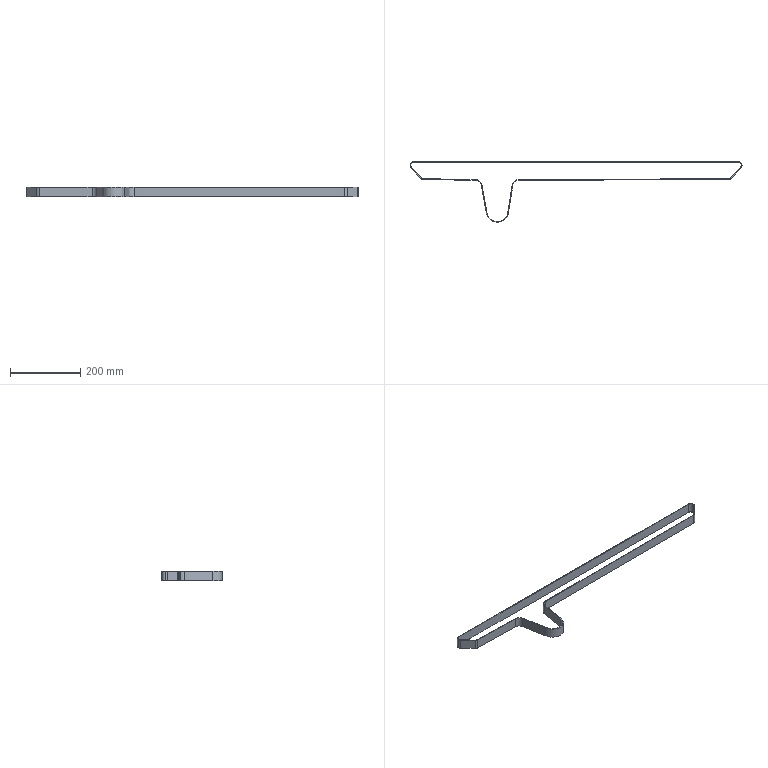Component | SolidWorks | --MA18S20041JR-SHuangGWBelt1-1 | 1 solid | 32 faces | box 946 x 172 x 28 mm | volume 118080 mm3 | cylinder 16 | plane 16 | commonest cylinder face diameters 16 x5 20 x5 30 x2 34 x2 64 x1 60 x1
build123d program:
from build123d import *

# Parameters (mm, degrees)
EXTRUDE_THIN1_DEPTH = 28


with BuildPart() as part:
    # Sketch1 → Extrude-Thin1 (new body)
    with BuildSketch(Plane.XY):
        with BuildLine():
            Line((170.069, -109.183), (163.702, -27.72))
            ThreePointArc((163.702, -27.72), (159.583, -18.516), (150.567, -14))
            Line((150.567, -14), (1.149, 4.256))
            ThreePointArc((1.149, 4.256), (-2.62, 5.511), (-5.603, 8.136))
            Line((-5.603, 8.136), (-30.416, 40.821))
            ThreePointArc((-30.416, 40.821), (-31.17, 51.763), (-21.436, 56.816))
            Line((-21.436, 56.816), (899.788, -37.114))
            ThreePointArc((899.788, -37.114), (908.302, -44.028), (905.354, -54.592))
            Line((905.354, -54.592), (874.455, -81.597))
            ThreePointArc((874.455, -81.597), (870.933, -83.588), (866.91, -84.021))
            Line((866.91, -84.021), (269.576, -26.131))
            ThreePointArc((269.576, -26.131), (259.577, -28.738), (253.636, -37.194))
            Line((253.636, -37.194), (232.89, -114.939))
            ThreePointArc((232.89, -114.939), (199.052, -138.556), (170.069, -109.183))
        make_face()
        with BuildLine():
            Line((172.063, -109.027), (165.696, -27.564))
            ThreePointArc((165.696, -27.564), (161.028, -17.133), (150.81, -12.014))
            Line((150.81, -12.014), (1.392, 6.241))
            ThreePointArc((1.392, 6.241), (-1.624, 7.246), (-4.01, 9.345))
            Line((-4.01, 9.345), (-28.823, 42.03))
            ThreePointArc((-28.823, 42.03), (-29.427, 50.784), (-21.639, 54.826))
            Line((-21.639, 54.826), (899.585, -39.104))
            ThreePointArc((899.585, -39.104), (906.396, -44.635), (904.038, -53.086))
            Line((904.038, -53.086), (873.139, -80.091))
            ThreePointArc((873.139, -80.091), (870.321, -81.684), (867.103, -82.03))
            Line((867.103, -82.03), (269.769, -24.141))
            ThreePointArc((269.769, -24.141), (258.436, -27.095), (251.704, -36.678))
            Line((251.704, -36.678), (230.958, -114.424))
            ThreePointArc((230.958, -114.424), (199.234, -136.564), (172.063, -109.027))
        make_face(mode=Mode.SUBTRACT)
    extrude(amount=EXTRUDE_THIN1_DEPTH)


solid = part.part

# Placed as in the assembly
solid = solid.moved(Location((-138.867, 52.35, 19), (0, 0, 5.822)))
STEP:
#1=CARTESIAN_POINT('',(-6.534,4.122,1.85));
#2=VERTEX_POINT('',#1);
#3=CARTESIAN_POINT('',(-6.847,3.775,1.85));
#4=VERTEX_POINT('',#3);
#5=CARTESIAN_POINT('',(-6.534,3.807,1.85));
#6=DIRECTION('',(0.,0.,1.));
#7=DIRECTION('',(0.9948,0.1014,0.));
#8=AXIS2_PLACEMENT_3D('',#5,#6,#7);
#9=CIRCLE('',#8,0.315);
#10=EDGE_CURVE('',#2,#4,#9,.T.);
#11=ORIENTED_EDGE('',*,*,#10,.T.);
#12=CARTESIAN_POINT('',(-6.847,3.775,0.748));
#13=VERTEX_POINT('',#12);
#14=CARTESIAN_POINT('',(-6.847,3.775,1.85));
#15=DIRECTION('',(0.,0.,-1.));
#16=VECTOR('',#15,39.37);
#17=LINE('',#14,#16);
#18=EDGE_CURVE('',#4,#13,#17,.T.);
#19=ORIENTED_EDGE('',*,*,#18,.T.);
#20=CARTESIAN_POINT('',(-6.534,4.122,0.748));
#21=VERTEX_POINT('',#20);
#22=CARTESIAN_POINT('',(-6.534,3.807,0.748));
#23=DIRECTION('',(0.,0.,1.));
#24=DIRECTION('',(0.9948,0.1014,0.));
#25=AXIS2_PLACEMENT_3D('',#22,#23,#24);
#26=CIRCLE('',#25,0.315);
#27=EDGE_CURVE('',#21,#13,#26,.T.);
#28=ORIENTED_EDGE('',*,*,#27,.F.);
#29=CARTESIAN_POINT('',(-6.534,4.122,1.85));
#30=DIRECTION('',(0.,0.,-1.));
#31=VECTOR('',#30,39.37);
#32=LINE('',#29,#31);
#33=EDGE_CURVE('',#2,#21,#32,.T.);
#34=ORIENTED_EDGE('',*,*,#33,.F.);
#35=EDGE_LOOP('',(#11,#19,#28,#34));
#36=FACE_OUTER_BOUND('',#35,.T.);
#37=CARTESIAN_POINT('',(-6.534,3.807,1.85));
#38=DIRECTION('',(0.,0.,-1.));
#39=DIRECTION('',(-0.9948,-0.1014,0.));
#40=AXIS2_PLACEMENT_3D('',#37,#38,#39);
#41=CYLINDRICAL_SURFACE('',#40,0.315);
#42=ADVANCED_FACE('',(#36),#41,.F.);
#43=CARTESIAN_POINT('',(-6.925,3.767,1.85));
#44=VERTEX_POINT('',#43);
#45=CARTESIAN_POINT('',(-6.822,3.538,1.85));
#46=VERTEX_POINT('',#45);
#47=CARTESIAN_POINT('',(-6.534,3.807,1.85));
#48=DIRECTION('',(0.,0.,1.));
#49=DIRECTION('',(0.9948,0.1014,0.));
#50=AXIS2_PLACEMENT_3D('',#47,#48,#49);
#51=CIRCLE('',#50,0.3937);
#52=EDGE_CURVE('',#44,#46,#51,.T.);
#53=ORIENTED_EDGE('',*,*,#52,.F.);
#54=CARTESIAN_POINT('',(-6.925,3.767,0.748));
#55=VERTEX_POINT('',#54);
#56=CARTESIAN_POINT('',(-6.925,3.767,1.85));
#57=DIRECTION('',(0.,0.,-1.));
#58=VECTOR('',#57,39.37);
#59=LINE('',#56,#58);
#60=EDGE_CURVE('',#44,#55,#59,.T.);
#61=ORIENTED_EDGE('',*,*,#60,.T.);
#62=CARTESIAN_POINT('',(-6.822,3.538,0.748));
#63=VERTEX_POINT('',#62);
#64=CARTESIAN_POINT('',(-6.534,3.807,0.748));
#65=DIRECTION('',(0.,0.,1.));
#66=DIRECTION('',(0.9948,0.1014,0.));
#67=AXIS2_PLACEMENT_3D('',#64,#65,#66);
#68=CIRCLE('',#67,0.3937);
#69=EDGE_CURVE('',#55,#63,#68,.T.);
#70=ORIENTED_EDGE('',*,*,#69,.T.);
#71=CARTESIAN_POINT('',(-6.822,3.538,1.85));
#72=DIRECTION('',(0.,0.,-1.));
#73=VECTOR('',#72,39.37);
#74=LINE('',#71,#73);
#75=EDGE_CURVE('',#46,#63,#74,.T.);
#76=ORIENTED_EDGE('',*,*,#75,.F.);
#77=EDGE_LOOP('',(#53,#61,#70,#76));
#78=FACE_OUTER_BOUND('',#77,.T.);
#79=CARTESIAN_POINT('',(-6.534,3.807,1.85));
#80=DIRECTION('',(0.,0.,-1.));
#81=DIRECTION('',(-0.9948,-0.1014,0.));
#82=AXIS2_PLACEMENT_3D('',#79,#80,#81);
#83=CYLINDRICAL_SURFACE('',#82,0.3937);
#84=ADVANCED_FACE('',(#78),#83,.T.);
#85=CARTESIAN_POINT('',(30.211,3.538,1.85));
#86=VERTEX_POINT('',#85);
#87=CARTESIAN_POINT('',(29.923,4.201,1.85));
#88=VERTEX_POINT('',#87);
#89=CARTESIAN_POINT('',(29.923,3.807,1.85));
#90=DIRECTION('',(0.,0.,1.));
#91=DIRECTION('',(0.9948,0.1014,0.));
#92=AXIS2_PLACEMENT_3D('',#89,#90,#91);
#93=CIRCLE('',#92,0.3937);
#94=EDGE_CURVE('',#86,#88,#93,.T.);
#95=ORIENTED_EDGE('',*,*,#94,.T.);
#96=CARTESIAN_POINT('',(-6.534,4.201,1.85));
#97=VERTEX_POINT('',#96);
#98=CARTESIAN_POINT('',(-6.534,4.201,1.85));
#99=DIRECTION('',(-1.,0.,0.));
#100=VECTOR('',#99,39.37);
#101=LINE('',#98,#100);
#102=EDGE_CURVE('',#88,#97,#101,.T.);
#103=ORIENTED_EDGE('',*,*,#102,.T.);
#104=CARTESIAN_POINT('',(-6.534,3.807,1.85));
#105=DIRECTION('',(0.,0.,1.));
#106=DIRECTION('',(0.9948,0.1014,0.));
#107=AXIS2_PLACEMENT_3D('',#104,#105,#106);
#108=CIRCLE('',#107,0.3937);
#109=EDGE_CURVE('',#97,#44,#108,.T.);
#110=ORIENTED_EDGE('',*,*,#109,.T.);
#111=ORIENTED_EDGE('',*,*,#52,.T.);
#112=CARTESIAN_POINT('',(-5.719,2.357,1.85));
#113=VERTEX_POINT('',#112);
#114=CARTESIAN_POINT('',(-5.719,2.357,1.85));
#115=DIRECTION('',(0.6823,-0.7311,0.));
#116=VECTOR('',#115,39.37);
#117=LINE('',#114,#116);
#118=EDGE_CURVE('',#46,#113,#117,.T.);
#119=ORIENTED_EDGE('',*,*,#118,.T.);
#120=CARTESIAN_POINT('',(-5.439,2.232,1.85));
#121=VERTEX_POINT('',#120);
#122=CARTESIAN_POINT('',(-5.431,2.626,1.85));
#123=DIRECTION('',(0.,0.,1.));
#124=DIRECTION('',(0.9948,0.1014,0.));
#125=AXIS2_PLACEMENT_3D('',#122,#123,#124);
#126=CIRCLE('',#125,0.3937);
#127=EDGE_CURVE('',#113,#121,#126,.T.);
#128=ORIENTED_EDGE('',*,*,#127,.T.);
#129=CARTESIAN_POINT('',(0.486,2.114,1.85));
#130=VERTEX_POINT('',#129);
#131=CARTESIAN_POINT('',(-5.439,2.232,1.85));
#132=DIRECTION('',(0.9998,-0.01996,0.));
#133=VECTOR('',#132,39.37);
#134=LINE('',#131,#133);
#135=EDGE_CURVE('',#121,#130,#134,.T.);
#136=ORIENTED_EDGE('',*,*,#135,.T.);
#137=CARTESIAN_POINT('',(1.055,1.629,1.85));
#138=VERTEX_POINT('',#137);
#139=CARTESIAN_POINT('',(0.4742,1.524,1.85));
#140=DIRECTION('',(0.,0.,-1.));
#141=DIRECTION('',(0.9948,0.1014,0.));
#142=AXIS2_PLACEMENT_3D('',#139,#140,#141);
#143=CIRCLE('',#142,0.5906);
#144=EDGE_CURVE('',#130,#138,#143,.T.);
#145=ORIENTED_EDGE('',*,*,#144,.T.);
#146=CARTESIAN_POINT('',(1.63,-1.536,1.85));
#147=VERTEX_POINT('',#146);
#148=CARTESIAN_POINT('',(1.63,-1.536,1.85));
#149=DIRECTION('',(0.1786,-0.9839,0.));
#150=VECTOR('',#149,39.37);
#151=LINE('',#148,#150);
#152=EDGE_CURVE('',#138,#147,#151,.T.);
#153=ORIENTED_EDGE('',*,*,#152,.T.);
#154=CARTESIAN_POINT('',(4.113,-1.511,1.85));
#155=VERTEX_POINT('',#154);
#156=CARTESIAN_POINT('',(2.869,-1.311,1.85));
#157=DIRECTION('',(0.,0.,1.));
#158=DIRECTION('',(0.9948,0.1014,0.));
#159=AXIS2_PLACEMENT_3D('',#156,#157,#158);
#160=CIRCLE('',#159,1.26);
#161=EDGE_CURVE('',#147,#155,#160,.T.);
#162=ORIENTED_EDGE('',*,*,#161,.T.);
#163=CARTESIAN_POINT('',(4.615,1.617,1.85));
#164=VERTEX_POINT('',#163);
#165=CARTESIAN_POINT('',(4.615,1.617,1.85));
#166=DIRECTION('',(0.1585,0.9874,0.));
#167=VECTOR('',#166,39.37);
#168=LINE('',#165,#167);
#169=EDGE_CURVE('',#155,#164,#168,.T.);
#170=ORIENTED_EDGE('',*,*,#169,.T.);
#171=CARTESIAN_POINT('',(5.196,2.114,1.85));
#172=VERTEX_POINT('',#171);
#173=CARTESIAN_POINT('',(5.199,1.524,1.85));
#174=DIRECTION('',(0.,0.,-1.));
#175=DIRECTION('',(0.9948,0.1014,0.));
#176=AXIS2_PLACEMENT_3D('',#173,#174,#175);
#177=CIRCLE('',#176,0.5906);
#178=EDGE_CURVE('',#164,#172,#177,.T.);
#179=ORIENTED_EDGE('',*,*,#178,.T.);
#180=CARTESIAN_POINT('',(28.823,2.232,1.85));
#181=VERTEX_POINT('',#180);
#182=CARTESIAN_POINT('',(28.823,2.232,1.85));
#183=DIRECTION('',(1.,0.004999,0.));
#184=VECTOR('',#183,39.37);
#185=LINE('',#182,#184);
#186=EDGE_CURVE('',#172,#181,#185,.T.);
#187=ORIENTED_EDGE('',*,*,#186,.T.);
#188=CARTESIAN_POINT('',(29.108,2.357,1.85));
#189=VERTEX_POINT('',#188);
#190=CARTESIAN_POINT('',(28.821,2.626,1.85));
#191=DIRECTION('',(0.,0.,1.));
#192=DIRECTION('',(0.9948,0.1014,0.));
#193=AXIS2_PLACEMENT_3D('',#190,#191,#192);
#194=CIRCLE('',#193,0.3937);
#195=EDGE_CURVE('',#181,#189,#194,.T.);
#196=ORIENTED_EDGE('',*,*,#195,.T.);
#197=CARTESIAN_POINT('',(30.211,3.538,1.85));
#198=DIRECTION('',(0.6823,0.7311,0.));
#199=VECTOR('',#198,39.37);
#200=LINE('',#197,#199);
#201=EDGE_CURVE('',#189,#86,#200,.T.);
#202=ORIENTED_EDGE('',*,*,#201,.T.);
#203=EDGE_LOOP('',(#95,#103,#110,#111,#119,#128,#136,#145,#153,#162,#170,#179,#187,#196,#202));
#204=FACE_OUTER_BOUND('',#203,.T.);
#205=CARTESIAN_POINT('',(29.923,4.122,1.85));
#206=VERTEX_POINT('',#205);
#207=CARTESIAN_POINT('',(-6.534,4.122,1.85));
#208=DIRECTION('',(-1.,0.,0.));
#209=VECTOR('',#208,39.37);
#210=LINE('',#207,#209);
#211=EDGE_CURVE('',#206,#2,#210,.T.);
#212=ORIENTED_EDGE('',*,*,#211,.F.);
#213=CARTESIAN_POINT('',(30.153,3.592,1.85));
#214=VERTEX_POINT('',#213);
#215=CARTESIAN_POINT('',(29.923,3.807,1.85));
#216=DIRECTION('',(0.,0.,1.));
#217=DIRECTION('',(0.9948,0.1014,0.));
#218=AXIS2_PLACEMENT_3D('',#215,#216,#217);
#219=CIRCLE('',#218,0.315);
#220=EDGE_CURVE('',#214,#206,#219,.T.);
#221=ORIENTED_EDGE('',*,*,#220,.F.);
#222=CARTESIAN_POINT('',(29.051,2.411,1.85));
#223=VERTEX_POINT('',#222);
#224=CARTESIAN_POINT('',(30.153,3.592,1.85));
#225=DIRECTION('',(0.6823,0.7311,0.));
#226=VECTOR('',#225,39.37);
#227=LINE('',#224,#226);
#228=EDGE_CURVE('',#223,#214,#227,.T.);
#229=ORIENTED_EDGE('',*,*,#228,.F.);
#230=CARTESIAN_POINT('',(28.822,2.311,1.85));
#231=VERTEX_POINT('',#230);
#232=CARTESIAN_POINT('',(28.821,2.626,1.85));
#233=DIRECTION('',(0.,0.,1.));
#234=DIRECTION('',(0.9948,0.1014,0.));
#235=AXIS2_PLACEMENT_3D('',#232,#233,#234);
#236=CIRCLE('',#235,0.315);
#237=EDGE_CURVE('',#231,#223,#236,.T.);
#238=ORIENTED_EDGE('',*,*,#237,.F.);
#239=CARTESIAN_POINT('',(5.195,2.193,1.85));
#240=VERTEX_POINT('',#239);
#241=CARTESIAN_POINT('',(28.822,2.311,1.85));
#242=DIRECTION('',(1.,0.004999,0.));
#243=VECTOR('',#242,39.37);
#244=LINE('',#241,#243);
#245=EDGE_CURVE('',#240,#231,#244,.T.);
#246=ORIENTED_EDGE('',*,*,#245,.F.);
#247=CARTESIAN_POINT('',(4.538,1.63,1.85));
#248=VERTEX_POINT('',#247);
#249=CARTESIAN_POINT('',(5.199,1.524,1.85));
#250=DIRECTION('',(0.,0.,-1.));
#251=DIRECTION('',(0.9948,0.1014,0.));
#252=AXIS2_PLACEMENT_3D('',#249,#250,#251);
#253=CIRCLE('',#252,0.6693);
#254=EDGE_CURVE('',#248,#240,#253,.T.);
#255=ORIENTED_EDGE('',*,*,#254,.F.);
#256=CARTESIAN_POINT('',(4.036,-1.498,1.85));
#257=VERTEX_POINT('',#256);
#258=CARTESIAN_POINT('',(4.538,1.63,1.85));
#259=DIRECTION('',(0.1585,0.9874,0.));
#260=VECTOR('',#259,39.37);
#261=LINE('',#258,#260);
#262=EDGE_CURVE('',#257,#248,#261,.T.);
#263=ORIENTED_EDGE('',*,*,#262,.F.);
#264=CARTESIAN_POINT('',(1.707,-1.522,1.85));
#265=VERTEX_POINT('',#264);
#266=CARTESIAN_POINT('',(2.869,-1.311,1.85));
#267=DIRECTION('',(0.,0.,1.));
#268=DIRECTION('',(0.9948,0.1014,0.));
#269=AXIS2_PLACEMENT_3D('',#266,#267,#268);
#270=CIRCLE('',#269,1.181);
#271=EDGE_CURVE('',#265,#257,#270,.T.);
#272=ORIENTED_EDGE('',*,*,#271,.F.);
#273=CARTESIAN_POINT('',(1.133,1.643,1.85));
#274=VERTEX_POINT('',#273);
#275=CARTESIAN_POINT('',(1.707,-1.522,1.85));
#276=DIRECTION('',(0.1786,-0.9839,0.));
#277=VECTOR('',#276,39.37);
#278=LINE('',#275,#277);
#279=EDGE_CURVE('',#274,#265,#278,.T.);
#280=ORIENTED_EDGE('',*,*,#279,.F.);
#281=CARTESIAN_POINT('',(0.4875,2.193,1.85));
#282=VERTEX_POINT('',#281);
#283=CARTESIAN_POINT('',(0.4742,1.524,1.85));
#284=DIRECTION('',(0.,0.,-1.));
#285=DIRECTION('',(0.9948,0.1014,0.));
#286=AXIS2_PLACEMENT_3D('',#283,#284,#285);
#287=CIRCLE('',#286,0.6693);
#288=EDGE_CURVE('',#282,#274,#287,.T.);
#289=ORIENTED_EDGE('',*,*,#288,.F.);
#290=CARTESIAN_POINT('',(-5.438,2.311,1.85));
#291=VERTEX_POINT('',#290);
#292=CARTESIAN_POINT('',(-5.438,2.311,1.85));
#293=DIRECTION('',(0.9998,-0.01996,0.));
#294=VECTOR('',#293,39.37);
#295=LINE('',#292,#294);
#296=EDGE_CURVE('',#291,#282,#295,.T.);
#297=ORIENTED_EDGE('',*,*,#296,.F.);
#298=CARTESIAN_POINT('',(-5.662,2.411,1.85));
#299=VERTEX_POINT('',#298);
#300=CARTESIAN_POINT('',(-5.431,2.626,1.85));
#301=DIRECTION('',(0.,0.,1.));
#302=DIRECTION('',(0.9948,0.1014,0.));
#303=AXIS2_PLACEMENT_3D('',#300,#301,#302);
#304=CIRCLE('',#303,0.315);
#305=EDGE_CURVE('',#299,#291,#304,.T.);
#306=ORIENTED_EDGE('',*,*,#305,.F.);
#307=CARTESIAN_POINT('',(-6.764,3.592,1.85));
#308=VERTEX_POINT('',#307);
#309=CARTESIAN_POINT('',(-5.662,2.411,1.85));
#310=DIRECTION('',(0.6823,-0.7311,0.));
#311=VECTOR('',#310,39.37);
#312=LINE('',#309,#311);
#313=EDGE_CURVE('',#308,#299,#312,.T.);
#314=ORIENTED_EDGE('',*,*,#313,.F.);
#315=CARTESIAN_POINT('',(-6.534,3.807,1.85));
#316=DIRECTION('',(0.,0.,1.));
#317=DIRECTION('',(0.9948,0.1014,0.));
#318=AXIS2_PLACEMENT_3D('',#315,#316,#317);
#319=CIRCLE('',#318,0.315);
#320=EDGE_CURVE('',#4,#308,#319,.T.);
#321=ORIENTED_EDGE('',*,*,#320,.F.);
#322=ORIENTED_EDGE('',*,*,#10,.F.);
#323=EDGE_LOOP('',(#212,#221,#229,#238,#246,#255,#263,#272,#280,#289,#297,#306,#314,#321,#322));
#324=FACE_BOUND('',#323,.T.);
#325=CARTESIAN_POINT('',(29.923,3.807,1.85));
#326=DIRECTION('',(0.,0.,1.));
#327=DIRECTION('',(0.9948,0.1014,0.));
#328=AXIS2_PLACEMENT_3D('',#325,#326,#327);
#329=PLANE('',#328);
#330=ADVANCED_FACE('',(#204,#324),#329,.T.);
#331=CARTESIAN_POINT('',(30.211,3.538,0.748));
#332=VERTEX_POINT('',#331);
#333=CARTESIAN_POINT('',(29.923,4.201,0.748));
#334=VERTEX_POINT('',#333);
#335=CARTESIAN_POINT('',(29.923,3.807,0.748));
#336=DIRECTION('',(0.,0.,1.));
#337=DIRECTION('',(0.9948,0.1014,0.));
#338=AXIS2_PLACEMENT_3D('',#335,#336,#337);
#339=CIRCLE('',#338,0.3937);
#340=EDGE_CURVE('',#332,#334,#339,.T.);
#341=ORIENTED_EDGE('',*,*,#340,.F.);
#342=CARTESIAN_POINT('',(29.108,2.357,0.748));
#343=VERTEX_POINT('',#342);
#344=CARTESIAN_POINT('',(30.211,3.538,0.748));
#345=DIRECTION('',(0.6823,0.7311,0.));
#346=VECTOR('',#345,39.37);
#347=LINE('',#344,#346);
#348=EDGE_CURVE('',#343,#332,#347,.T.);
#349=ORIENTED_EDGE('',*,*,#348,.F.);
#350=CARTESIAN_POINT('',(28.823,2.232,0.748));
#351=VERTEX_POINT('',#350);
#352=CARTESIAN_POINT('',(28.821,2.626,0.748));
#353=DIRECTION('',(0.,0.,1.));
#354=DIRECTION('',(0.9948,0.1014,0.));
#355=AXIS2_PLACEMENT_3D('',#352,#353,#354);
#356=CIRCLE('',#355,0.3937);
#357=EDGE_CURVE('',#351,#343,#356,.T.);
#358=ORIENTED_EDGE('',*,*,#357,.F.);
#359=CARTESIAN_POINT('',(5.196,2.114,0.748));
#360=VERTEX_POINT('',#359);
#361=CARTESIAN_POINT('',(28.823,2.232,0.748));
#362=DIRECTION('',(1.,0.004999,0.));
#363=VECTOR('',#362,39.37);
#364=LINE('',#361,#363);
#365=EDGE_CURVE('',#360,#351,#364,.T.);
#366=ORIENTED_EDGE('',*,*,#365,.F.);
#367=CARTESIAN_POINT('',(4.615,1.617,0.748));
#368=VERTEX_POINT('',#367);
#369=CARTESIAN_POINT('',(5.199,1.524,0.748));
#370=DIRECTION('',(0.,0.,-1.));
#371=DIRECTION('',(0.9948,0.1014,0.));
#372=AXIS2_PLACEMENT_3D('',#369,#370,#371);
#373=CIRCLE('',#372,0.5906);
#374=EDGE_CURVE('',#368,#360,#373,.T.);
#375=ORIENTED_EDGE('',*,*,#374,.F.);
#376=CARTESIAN_POINT('',(4.113,-1.511,0.748));
#377=VERTEX_POINT('',#376);
#378=CARTESIAN_POINT('',(4.615,1.617,0.748));
#379=DIRECTION('',(0.1585,0.9874,0.));
#380=VECTOR('',#379,39.37);
#381=LINE('',#378,#380);
#382=EDGE_CURVE('',#377,#368,#381,.T.);
#383=ORIENTED_EDGE('',*,*,#382,.F.);
#384=CARTESIAN_POINT('',(1.63,-1.536,0.748));
#385=VERTEX_POINT('',#384);
#386=CARTESIAN_POINT('',(2.869,-1.311,0.748));
#387=DIRECTION('',(0.,0.,1.));
#388=DIRECTION('',(0.9948,0.1014,0.));
#389=AXIS2_PLACEMENT_3D('',#386,#387,#388);
#390=CIRCLE('',#389,1.26);
#391=EDGE_CURVE('',#385,#377,#390,.T.);
#392=ORIENTED_EDGE('',*,*,#391,.F.);
#393=CARTESIAN_POINT('',(1.055,1.629,0.748));
#394=VERTEX_POINT('',#393);
#395=CARTESIAN_POINT('',(1.63,-1.536,0.748));
#396=DIRECTION('',(0.1786,-0.9839,0.));
#397=VECTOR('',#396,39.37);
#398=LINE('',#395,#397);
#399=EDGE_CURVE('',#394,#385,#398,.T.);
#400=ORIENTED_EDGE('',*,*,#399,.F.);
#401=CARTESIAN_POINT('',(0.486,2.114,0.748));
#402=VERTEX_POINT('',#401);
#403=CARTESIAN_POINT('',(0.4742,1.524,0.748));
#404=DIRECTION('',(0.,0.,-1.));
#405=DIRECTION('',(0.9948,0.1014,0.));
#406=AXIS2_PLACEMENT_3D('',#403,#404,#405);
#407=CIRCLE('',#406,0.5906);
#408=EDGE_CURVE('',#402,#394,#407,.T.);
#409=ORIENTED_EDGE('',*,*,#408,.F.);
#410=CARTESIAN_POINT('',(-5.439,2.232,0.748));
#411=VERTEX_POINT('',#410);
#412=CARTESIAN_POINT('',(-5.439,2.232,0.748));
#413=DIRECTION('',(0.9998,-0.01996,0.));
#414=VECTOR('',#413,39.37);
#415=LINE('',#412,#414);
#416=EDGE_CURVE('',#411,#402,#415,.T.);
#417=ORIENTED_EDGE('',*,*,#416,.F.);
#418=CARTESIAN_POINT('',(-5.719,2.357,0.748));
#419=VERTEX_POINT('',#418);
#420=CARTESIAN_POINT('',(-5.431,2.626,0.748));
#421=DIRECTION('',(0.,0.,1.));
#422=DIRECTION('',(0.9948,0.1014,0.));
#423=AXIS2_PLACEMENT_3D('',#420,#421,#422);
#424=CIRCLE('',#423,0.3937);
#425=EDGE_CURVE('',#419,#411,#424,.T.);
#426=ORIENTED_EDGE('',*,*,#425,.F.);
#427=CARTESIAN_POINT('',(-5.719,2.357,0.748));
#428=DIRECTION('',(0.6823,-0.7311,0.));
#429=VECTOR('',#428,39.37);
#430=LINE('',#427,#429);
#431=EDGE_CURVE('',#63,#419,#430,.T.);
#432=ORIENTED_EDGE('',*,*,#431,.F.);
#433=ORIENTED_EDGE('',*,*,#69,.F.);
#434=CARTESIAN_POINT('',(-6.534,4.201,0.748));
#435=VERTEX_POINT('',#434);
#436=CARTESIAN_POINT('',(-6.534,3.807,0.748));
#437=DIRECTION('',(0.,0.,1.));
#438=DIRECTION('',(0.9948,0.1014,0.));
#439=AXIS2_PLACEMENT_3D('',#436,#437,#438);
#440=CIRCLE('',#439,0.3937);
#441=EDGE_CURVE('',#435,#55,#440,.T.);
#442=ORIENTED_EDGE('',*,*,#441,.F.);
#443=CARTESIAN_POINT('',(-6.534,4.201,0.748));
#444=DIRECTION('',(-1.,0.,0.));
#445=VECTOR('',#444,39.37);
#446=LINE('',#443,#445);
#447=EDGE_CURVE('',#334,#435,#446,.T.);
#448=ORIENTED_EDGE('',*,*,#447,.F.);
#449=EDGE_LOOP('',(#341,#349,#358,#366,#375,#383,#392,#400,#409,#417,#426,#432,#433,#442,#448));
#450=FACE_OUTER_BOUND('',#449,.T.);
#451=CARTESIAN_POINT('',(30.153,3.592,0.748));
#452=VERTEX_POINT('',#451);
#453=CARTESIAN_POINT('',(29.923,4.122,0.748));
#454=VERTEX_POINT('',#453);
#455=CARTESIAN_POINT('',(29.923,3.807,0.748));
#456=DIRECTION('',(0.,0.,1.));
#457=DIRECTION('',(0.9948,0.1014,0.));
#458=AXIS2_PLACEMENT_3D('',#455,#456,#457);
#459=CIRCLE('',#458,0.315);
#460=EDGE_CURVE('',#452,#454,#459,.T.);
#461=ORIENTED_EDGE('',*,*,#460,.T.);
#462=CARTESIAN_POINT('',(-6.534,4.122,0.748));
#463=DIRECTION('',(-1.,0.,0.));
#464=VECTOR('',#463,39.37);
#465=LINE('',#462,#464);
#466=EDGE_CURVE('',#454,#21,#465,.T.);
#467=ORIENTED_EDGE('',*,*,#466,.T.);
#468=ORIENTED_EDGE('',*,*,#27,.T.);
#469=CARTESIAN_POINT('',(-6.764,3.592,0.748));
#470=VERTEX_POINT('',#469);
#471=CARTESIAN_POINT('',(-6.534,3.807,0.748));
#472=DIRECTION('',(0.,0.,1.));
#473=DIRECTION('',(0.9948,0.1014,0.));
#474=AXIS2_PLACEMENT_3D('',#471,#472,#473);
#475=CIRCLE('',#474,0.315);
#476=EDGE_CURVE('',#13,#470,#475,.T.);
#477=ORIENTED_EDGE('',*,*,#476,.T.);
#478=CARTESIAN_POINT('',(-5.662,2.411,0.748));
#479=VERTEX_POINT('',#478);
#480=CARTESIAN_POINT('',(-5.662,2.411,0.748));
#481=DIRECTION('',(0.6823,-0.7311,0.));
#482=VECTOR('',#481,39.37);
#483=LINE('',#480,#482);
#484=EDGE_CURVE('',#470,#479,#483,.T.);
#485=ORIENTED_EDGE('',*,*,#484,.T.);
#486=CARTESIAN_POINT('',(-5.438,2.311,0.748));
#487=VERTEX_POINT('',#486);
#488=CARTESIAN_POINT('',(-5.431,2.626,0.748));
#489=DIRECTION('',(0.,0.,1.));
#490=DIRECTION('',(0.9948,0.1014,0.));
#491=AXIS2_PLACEMENT_3D('',#488,#489,#490);
#492=CIRCLE('',#491,0.315);
#493=EDGE_CURVE('',#479,#487,#492,.T.);
#494=ORIENTED_EDGE('',*,*,#493,.T.);
#495=CARTESIAN_POINT('',(0.4875,2.193,0.748));
#496=VERTEX_POINT('',#495);
#497=CARTESIAN_POINT('',(-5.438,2.311,0.748));
#498=DIRECTION('',(0.9998,-0.01996,0.));
#499=VECTOR('',#498,39.37);
#500=LINE('',#497,#499);
#501=EDGE_CURVE('',#487,#496,#500,.T.);
#502=ORIENTED_EDGE('',*,*,#501,.T.);
#503=CARTESIAN_POINT('',(1.133,1.643,0.748));
#504=VERTEX_POINT('',#503);
#505=CARTESIAN_POINT('',(0.4742,1.524,0.748));
#506=DIRECTION('',(0.,0.,-1.));
#507=DIRECTION('',(0.9948,0.1014,0.));
#508=AXIS2_PLACEMENT_3D('',#505,#506,#507);
#509=CIRCLE('',#508,0.6693);
#510=EDGE_CURVE('',#496,#504,#509,.T.);
#511=ORIENTED_EDGE('',*,*,#510,.T.);
#512=CARTESIAN_POINT('',(1.707,-1.522,0.748));
#513=VERTEX_POINT('',#512);
#514=CARTESIAN_POINT('',(1.707,-1.522,0.748));
#515=DIRECTION('',(0.1786,-0.9839,0.));
#516=VECTOR('',#515,39.37);
#517=LINE('',#514,#516);
#518=EDGE_CURVE('',#504,#513,#517,.T.);
#519=ORIENTED_EDGE('',*,*,#518,.T.);
#520=CARTESIAN_POINT('',(4.036,-1.498,0.748));
#521=VERTEX_POINT('',#520);
#522=CARTESIAN_POINT('',(2.869,-1.311,0.748));
#523=DIRECTION('',(0.,0.,1.));
#524=DIRECTION('',(0.9948,0.1014,0.));
#525=AXIS2_PLACEMENT_3D('',#522,#523,#524);
#526=CIRCLE('',#525,1.181);
#527=EDGE_CURVE('',#513,#521,#526,.T.);
#528=ORIENTED_EDGE('',*,*,#527,.T.);
#529=CARTESIAN_POINT('',(4.538,1.63,0.748));
#530=VERTEX_POINT('',#529);
#531=CARTESIAN_POINT('',(4.538,1.63,0.748));
#532=DIRECTION('',(0.1585,0.9874,0.));
#533=VECTOR('',#532,39.37);
#534=LINE('',#531,#533);
#535=EDGE_CURVE('',#521,#530,#534,.T.);
#536=ORIENTED_EDGE('',*,*,#535,.T.);
#537=CARTESIAN_POINT('',(5.195,2.193,0.748));
#538=VERTEX_POINT('',#537);
#539=CARTESIAN_POINT('',(5.199,1.524,0.748));
#540=DIRECTION('',(0.,0.,-1.));
#541=DIRECTION('',(0.9948,0.1014,0.));
#542=AXIS2_PLACEMENT_3D('',#539,#540,#541);
#543=CIRCLE('',#542,0.6693);
#544=EDGE_CURVE('',#530,#538,#543,.T.);
#545=ORIENTED_EDGE('',*,*,#544,.T.);
#546=CARTESIAN_POINT('',(28.822,2.311,0.748));
#547=VERTEX_POINT('',#546);
#548=CARTESIAN_POINT('',(28.822,2.311,0.748));
#549=DIRECTION('',(1.,0.004999,0.));
#550=VECTOR('',#549,39.37);
#551=LINE('',#548,#550);
#552=EDGE_CURVE('',#538,#547,#551,.T.);
#553=ORIENTED_EDGE('',*,*,#552,.T.);
#554=CARTESIAN_POINT('',(29.051,2.411,0.748));
#555=VERTEX_POINT('',#554);
#556=CARTESIAN_POINT('',(28.821,2.626,0.748));
#557=DIRECTION('',(0.,0.,1.));
#558=DIRECTION('',(0.9948,0.1014,0.));
#559=AXIS2_PLACEMENT_3D('',#556,#557,#558);
#560=CIRCLE('',#559,0.315);
#561=EDGE_CURVE('',#547,#555,#560,.T.);
#562=ORIENTED_EDGE('',*,*,#561,.T.);
#563=CARTESIAN_POINT('',(30.153,3.592,0.748));
#564=DIRECTION('',(0.6823,0.7311,0.));
#565=VECTOR('',#564,39.37);
#566=LINE('',#563,#565);
#567=EDGE_CURVE('',#555,#452,#566,.T.);
#568=ORIENTED_EDGE('',*,*,#567,.T.);
#569=EDGE_LOOP('',(#461,#467,#468,#477,#485,#494,#502,#511,#519,#528,#536,#545,#553,#562,#568));
#570=FACE_BOUND('',#569,.T.);
#571=CARTESIAN_POINT('',(29.923,3.807,0.748));
#572=DIRECTION('',(0.,0.,1.));
#573=DIRECTION('',(0.9948,0.1014,0.));
#574=AXIS2_PLACEMENT_3D('',#571,#572,#573);
#575=PLANE('',#574);
#576=ADVANCED_FACE('',(#450,#570),#575,.F.);
#577=ORIENTED_EDGE('',*,*,#340,.T.);
#578=CARTESIAN_POINT('',(29.923,4.201,1.85));
#579=DIRECTION('',(0.,0.,-1.));
#580=VECTOR('',#579,39.37);
#581=LINE('',#578,#580);
#582=EDGE_CURVE('',#88,#334,#581,.T.);
#583=ORIENTED_EDGE('',*,*,#582,.F.);
#584=ORIENTED_EDGE('',*,*,#94,.F.);
#585=CARTESIAN_POINT('',(30.211,3.538,1.85));
#586=DIRECTION('',(0.,0.,-1.));
#587=VECTOR('',#586,39.37);
#588=LINE('',#585,#587);
#589=EDGE_CURVE('',#86,#332,#588,.T.);
#590=ORIENTED_EDGE('',*,*,#589,.T.);
#591=EDGE_LOOP('',(#577,#583,#584,#590));
#592=FACE_OUTER_BOUND('',#591,.T.);
#593=CARTESIAN_POINT('',(29.923,3.807,1.85));
#594=DIRECTION('',(0.,0.,-1.));
#595=DIRECTION('',(-0.9948,-0.1014,0.));
#596=AXIS2_PLACEMENT_3D('',#593,#594,#595);
#597=CYLINDRICAL_SURFACE('',#596,0.3937);
#598=ADVANCED_FACE('',(#592),#597,.T.);
#599=ORIENTED_EDGE('',*,*,#447,.T.);
#600=CARTESIAN_POINT('',(-6.534,4.201,1.85));
#601=DIRECTION('',(0.,0.,-1.));
#602=VECTOR('',#601,39.37);
#603=LINE('',#600,#602);
#604=EDGE_CURVE('',#97,#435,#603,.T.);
#605=ORIENTED_EDGE('',*,*,#604,.F.);
#606=ORIENTED_EDGE('',*,*,#102,.F.);
#607=ORIENTED_EDGE('',*,*,#582,.T.);
#608=EDGE_LOOP('',(#599,#605,#606,#607));
#609=FACE_OUTER_BOUND('',#608,.T.);
#610=CARTESIAN_POINT('',(-6.534,4.201,1.85));
#611=DIRECTION('',(-0.,-1.,0.));
#612=DIRECTION('',(1.,-0.,0.));
#613=AXIS2_PLACEMENT_3D('',#610,#611,#612);
#614=PLANE('',#613);
#615=ADVANCED_FACE('',(#609),#614,.F.);
#616=ORIENTED_EDGE('',*,*,#60,.F.);
#617=ORIENTED_EDGE('',*,*,#109,.F.);
#618=ORIENTED_EDGE('',*,*,#604,.T.);
#619=ORIENTED_EDGE('',*,*,#441,.T.);
#620=EDGE_LOOP('',(#616,#617,#618,#619));
#621=FACE_OUTER_BOUND('',#620,.T.);
#622=CARTESIAN_POINT('',(-6.534,3.807,1.85));
#623=DIRECTION('',(0.,0.,-1.));
#624=DIRECTION('',(-0.9948,-0.1014,0.));
#625=AXIS2_PLACEMENT_3D('',#622,#623,#624);
#626=CYLINDRICAL_SURFACE('',#625,0.3937);
#627=ADVANCED_FACE('',(#621),#626,.T.);
#628=ORIENTED_EDGE('',*,*,#431,.T.);
#629=CARTESIAN_POINT('',(-5.719,2.357,1.85));
#630=DIRECTION('',(0.,0.,-1.));
#631=VECTOR('',#630,39.37);
#632=LINE('',#629,#631);
#633=EDGE_CURVE('',#113,#419,#632,.T.);
#634=ORIENTED_EDGE('',*,*,#633,.F.);
#635=ORIENTED_EDGE('',*,*,#118,.F.);
#636=ORIENTED_EDGE('',*,*,#75,.T.);
#637=EDGE_LOOP('',(#628,#634,#635,#636));
#638=FACE_OUTER_BOUND('',#637,.T.);
#639=CARTESIAN_POINT('',(-5.719,2.357,1.85));
#640=DIRECTION('',(0.7311,0.6823,0.));
#641=DIRECTION('',(-0.6823,0.7311,0.));
#642=AXIS2_PLACEMENT_3D('',#639,#640,#641);
#643=PLANE('',#642);
#644=ADVANCED_FACE('',(#638),#643,.F.);
#645=ORIENTED_EDGE('',*,*,#425,.T.);
#646=CARTESIAN_POINT('',(-5.439,2.232,1.85));
#647=DIRECTION('',(0.,0.,-1.));
#648=VECTOR('',#647,39.37);
#649=LINE('',#646,#648);
#650=EDGE_CURVE('',#121,#411,#649,.T.);
#651=ORIENTED_EDGE('',*,*,#650,.F.);
#652=ORIENTED_EDGE('',*,*,#127,.F.);
#653=ORIENTED_EDGE('',*,*,#633,.T.);
#654=EDGE_LOOP('',(#645,#651,#652,#653));
#655=FACE_OUTER_BOUND('',#654,.T.);
#656=CARTESIAN_POINT('',(-5.431,2.626,1.85));
#657=DIRECTION('',(0.,0.,-1.));
#658=DIRECTION('',(-0.9948,-0.1014,0.));
#659=AXIS2_PLACEMENT_3D('',#656,#657,#658);
#660=CYLINDRICAL_SURFACE('',#659,0.3937);
#661=ADVANCED_FACE('',(#655),#660,.T.);
#662=ORIENTED_EDGE('',*,*,#416,.T.);
#663=CARTESIAN_POINT('',(0.486,2.114,1.85));
#664=DIRECTION('',(0.,0.,-1.));
#665=VECTOR('',#664,39.37);
#666=LINE('',#663,#665);
#667=EDGE_CURVE('',#130,#402,#666,.T.);
#668=ORIENTED_EDGE('',*,*,#667,.F.);
#669=ORIENTED_EDGE('',*,*,#135,.F.);
#670=ORIENTED_EDGE('',*,*,#650,.T.);
#671=EDGE_LOOP('',(#662,#668,#669,#670));
#672=FACE_OUTER_BOUND('',#671,.T.);
#673=CARTESIAN_POINT('',(-5.439,2.232,1.85));
#674=DIRECTION('',(0.01996,0.9998,0.));
#675=DIRECTION('',(-0.9998,0.01996,0.));
#676=AXIS2_PLACEMENT_3D('',#673,#674,#675);
#677=PLANE('',#676);
#678=ADVANCED_FACE('',(#672),#677,.F.);
#679=ORIENTED_EDGE('',*,*,#408,.T.);
#680=CARTESIAN_POINT('',(1.055,1.629,1.85));
#681=DIRECTION('',(0.,0.,-1.));
#682=VECTOR('',#681,39.37);
#683=LINE('',#680,#682);
#684=EDGE_CURVE('',#138,#394,#683,.T.);
#685=ORIENTED_EDGE('',*,*,#684,.F.);
#686=ORIENTED_EDGE('',*,*,#144,.F.);
#687=ORIENTED_EDGE('',*,*,#667,.T.);
#688=EDGE_LOOP('',(#679,#685,#686,#687));
#689=FACE_OUTER_BOUND('',#688,.T.);
#690=CARTESIAN_POINT('',(0.4742,1.524,1.85));
#691=DIRECTION('',(0.,0.,-1.));
#692=DIRECTION('',(-0.9948,-0.1014,0.));
#693=AXIS2_PLACEMENT_3D('',#690,#691,#692);
#694=CYLINDRICAL_SURFACE('',#693,0.5906);
#695=ADVANCED_FACE('',(#689),#694,.F.);
#696=ORIENTED_EDGE('',*,*,#399,.T.);
#697=CARTESIAN_POINT('',(1.63,-1.536,1.85));
#698=DIRECTION('',(0.,0.,-1.));
#699=VECTOR('',#698,39.37);
#700=LINE('',#697,#699);
#701=EDGE_CURVE('',#147,#385,#700,.T.);
#702=ORIENTED_EDGE('',*,*,#701,.F.);
#703=ORIENTED_EDGE('',*,*,#152,.F.);
#704=ORIENTED_EDGE('',*,*,#684,.T.);
#705=EDGE_LOOP('',(#696,#702,#703,#704));
#706=FACE_OUTER_BOUND('',#705,.T.);
#707=CARTESIAN_POINT('',(1.63,-1.536,1.85));
#708=DIRECTION('',(0.9839,0.1786,0.));
#709=DIRECTION('',(-0.1786,0.9839,0.));
#710=AXIS2_PLACEMENT_3D('',#707,#708,#709);
#711=PLANE('',#710);
#712=ADVANCED_FACE('',(#706),#711,.F.);
#713=ORIENTED_EDGE('',*,*,#391,.T.);
#714=CARTESIAN_POINT('',(4.113,-1.511,1.85));
#715=DIRECTION('',(0.,0.,-1.));
#716=VECTOR('',#715,39.37);
#717=LINE('',#714,#716);
#718=EDGE_CURVE('',#155,#377,#717,.T.);
#719=ORIENTED_EDGE('',*,*,#718,.F.);
#720=ORIENTED_EDGE('',*,*,#161,.F.);
#721=ORIENTED_EDGE('',*,*,#701,.T.);
#722=EDGE_LOOP('',(#713,#719,#720,#721));
#723=FACE_OUTER_BOUND('',#722,.T.);
#724=CARTESIAN_POINT('',(2.869,-1.311,1.85));
#725=DIRECTION('',(0.,0.,-1.));
#726=DIRECTION('',(-0.9948,-0.1014,0.));
#727=AXIS2_PLACEMENT_3D('',#724,#725,#726);
#728=CYLINDRICAL_SURFACE('',#727,1.26);
#729=ADVANCED_FACE('',(#723),#728,.T.);
#730=ORIENTED_EDGE('',*,*,#382,.T.);
#731=CARTESIAN_POINT('',(4.615,1.617,1.85));
#732=DIRECTION('',(0.,0.,-1.));
#733=VECTOR('',#732,39.37);
#734=LINE('',#731,#733);
#735=EDGE_CURVE('',#164,#368,#734,.T.);
#736=ORIENTED_EDGE('',*,*,#735,.F.);
#737=ORIENTED_EDGE('',*,*,#169,.F.);
#738=ORIENTED_EDGE('',*,*,#718,.T.);
#739=EDGE_LOOP('',(#730,#736,#737,#738));
#740=FACE_OUTER_BOUND('',#739,.T.);
#741=CARTESIAN_POINT('',(4.615,1.617,1.85));
#742=DIRECTION('',(-0.9874,0.1585,0.));
#743=DIRECTION('',(-0.1585,-0.9874,0.));
#744=AXIS2_PLACEMENT_3D('',#741,#742,#743);
#745=PLANE('',#744);
#746=ADVANCED_FACE('',(#740),#745,.F.);
#747=ORIENTED_EDGE('',*,*,#374,.T.);
#748=CARTESIAN_POINT('',(5.196,2.114,1.85));
#749=DIRECTION('',(0.,0.,-1.));
#750=VECTOR('',#749,39.37);
#751=LINE('',#748,#750);
#752=EDGE_CURVE('',#172,#360,#751,.T.);
#753=ORIENTED_EDGE('',*,*,#752,.F.);
#754=ORIENTED_EDGE('',*,*,#178,.F.);
#755=ORIENTED_EDGE('',*,*,#735,.T.);
#756=EDGE_LOOP('',(#747,#753,#754,#755));
#757=FACE_OUTER_BOUND('',#756,.T.);
#758=CARTESIAN_POINT('',(5.199,1.524,1.85));
#759=DIRECTION('',(0.,0.,-1.));
#760=DIRECTION('',(-0.9948,-0.1014,0.));
#761=AXIS2_PLACEMENT_3D('',#758,#759,#760);
#762=CYLINDRICAL_SURFACE('',#761,0.5906);
#763=ADVANCED_FACE('',(#757),#762,.F.);
#764=ORIENTED_EDGE('',*,*,#365,.T.);
#765=CARTESIAN_POINT('',(28.823,2.232,1.85));
#766=DIRECTION('',(0.,0.,-1.));
#767=VECTOR('',#766,39.37);
#768=LINE('',#765,#767);
#769=EDGE_CURVE('',#181,#351,#768,.T.);
#770=ORIENTED_EDGE('',*,*,#769,.F.);
#771=ORIENTED_EDGE('',*,*,#186,.F.);
#772=ORIENTED_EDGE('',*,*,#752,.T.);
#773=EDGE_LOOP('',(#764,#770,#771,#772));
#774=FACE_OUTER_BOUND('',#773,.T.);
#775=CARTESIAN_POINT('',(28.823,2.232,1.85));
#776=DIRECTION('',(-0.004999,1.,0.));
#777=DIRECTION('',(-1.,-0.004999,0.));
#778=AXIS2_PLACEMENT_3D('',#775,#776,#777);
#779=PLANE('',#778);
#780=ADVANCED_FACE('',(#774),#779,.F.);
#781=ORIENTED_EDGE('',*,*,#357,.T.);
#782=CARTESIAN_POINT('',(29.108,2.357,1.85));
#783=DIRECTION('',(0.,0.,-1.));
#784=VECTOR('',#783,39.37);
#785=LINE('',#782,#784);
#786=EDGE_CURVE('',#189,#343,#785,.T.);
#787=ORIENTED_EDGE('',*,*,#786,.F.);
#788=ORIENTED_EDGE('',*,*,#195,.F.);
#789=ORIENTED_EDGE('',*,*,#769,.T.);
#790=EDGE_LOOP('',(#781,#787,#788,#789));
#791=FACE_OUTER_BOUND('',#790,.T.);
#792=CARTESIAN_POINT('',(28.821,2.626,1.85));
#793=DIRECTION('',(0.,0.,-1.));
#794=DIRECTION('',(-0.9948,-0.1014,0.));
#795=AXIS2_PLACEMENT_3D('',#792,#793,#794);
#796=CYLINDRICAL_SURFACE('',#795,0.3937);
#797=ADVANCED_FACE('',(#791),#796,.T.);
#798=ORIENTED_EDGE('',*,*,#348,.T.);
#799=ORIENTED_EDGE('',*,*,#589,.F.);
#800=ORIENTED_EDGE('',*,*,#201,.F.);
#801=ORIENTED_EDGE('',*,*,#786,.T.);
#802=EDGE_LOOP('',(#798,#799,#800,#801));
#803=FACE_OUTER_BOUND('',#802,.T.);
#804=CARTESIAN_POINT('',(30.211,3.538,1.85));
#805=DIRECTION('',(-0.7311,0.6823,0.));
#806=DIRECTION('',(-0.6823,-0.7311,0.));
#807=AXIS2_PLACEMENT_3D('',#804,#805,#806);
#808=PLANE('',#807);
#809=ADVANCED_FACE('',(#803),#808,.F.);
#810=ORIENTED_EDGE('',*,*,#460,.F.);
#811=CARTESIAN_POINT('',(30.153,3.592,1.85));
#812=DIRECTION('',(0.,0.,-1.));
#813=VECTOR('',#812,39.37);
#814=LINE('',#811,#813);
#815=EDGE_CURVE('',#214,#452,#814,.T.);
#816=ORIENTED_EDGE('',*,*,#815,.F.);
#817=ORIENTED_EDGE('',*,*,#220,.T.);
#818=CARTESIAN_POINT('',(29.923,4.122,1.85));
#819=DIRECTION('',(0.,0.,-1.));
#820=VECTOR('',#819,39.37);
#821=LINE('',#818,#820);
#822=EDGE_CURVE('',#206,#454,#821,.T.);
#823=ORIENTED_EDGE('',*,*,#822,.T.);
#824=EDGE_LOOP('',(#810,#816,#817,#823));
#825=FACE_OUTER_BOUND('',#824,.T.);
#826=CARTESIAN_POINT('',(29.923,3.807,1.85));
#827=DIRECTION('',(0.,0.,-1.));
#828=DIRECTION('',(-0.9948,-0.1014,0.));
#829=AXIS2_PLACEMENT_3D('',#826,#827,#828);
#830=CYLINDRICAL_SURFACE('',#829,0.315);
#831=ADVANCED_FACE('',(#825),#830,.F.);
#832=ORIENTED_EDGE('',*,*,#466,.F.);
#833=ORIENTED_EDGE('',*,*,#822,.F.);
#834=ORIENTED_EDGE('',*,*,#211,.T.);
#835=ORIENTED_EDGE('',*,*,#33,.T.);
#836=EDGE_LOOP('',(#832,#833,#834,#835));
#837=FACE_OUTER_BOUND('',#836,.T.);
#838=CARTESIAN_POINT('',(-6.534,4.122,1.85));
#839=DIRECTION('',(-0.,-1.,0.));
#840=DIRECTION('',(1.,-0.,0.));
#841=AXIS2_PLACEMENT_3D('',#838,#839,#840);
#842=PLANE('',#841);
#843=ADVANCED_FACE('',(#837),#842,.T.);
#844=ORIENTED_EDGE('',*,*,#18,.F.);
#845=ORIENTED_EDGE('',*,*,#320,.T.);
#846=CARTESIAN_POINT('',(-6.764,3.592,1.85));
#847=DIRECTION('',(0.,0.,-1.));
#848=VECTOR('',#847,39.37);
#849=LINE('',#846,#848);
#850=EDGE_CURVE('',#308,#470,#849,.T.);
#851=ORIENTED_EDGE('',*,*,#850,.T.);
#852=ORIENTED_EDGE('',*,*,#476,.F.);
#853=EDGE_LOOP('',(#844,#845,#851,#852));
#854=FACE_OUTER_BOUND('',#853,.T.);
#855=CARTESIAN_POINT('',(-6.534,3.807,1.85));
#856=DIRECTION('',(0.,0.,-1.));
#857=DIRECTION('',(-0.9948,-0.1014,0.));
#858=AXIS2_PLACEMENT_3D('',#855,#856,#857);
#859=CYLINDRICAL_SURFACE('',#858,0.315);
#860=ADVANCED_FACE('',(#854),#859,.F.);
#861=ORIENTED_EDGE('',*,*,#484,.F.);
#862=ORIENTED_EDGE('',*,*,#850,.F.);
#863=ORIENTED_EDGE('',*,*,#313,.T.);
#864=CARTESIAN_POINT('',(-5.662,2.411,1.85));
#865=DIRECTION('',(0.,0.,-1.));
#866=VECTOR('',#865,39.37);
#867=LINE('',#864,#866);
#868=EDGE_CURVE('',#299,#479,#867,.T.);
#869=ORIENTED_EDGE('',*,*,#868,.T.);
#870=EDGE_LOOP('',(#861,#862,#863,#869));
#871=FACE_OUTER_BOUND('',#870,.T.);
#872=CARTESIAN_POINT('',(-5.662,2.411,1.85));
#873=DIRECTION('',(0.7311,0.6823,0.));
#874=DIRECTION('',(-0.6823,0.7311,0.));
#875=AXIS2_PLACEMENT_3D('',#872,#873,#874);
#876=PLANE('',#875);
#877=ADVANCED_FACE('',(#871),#876,.T.);
#878=ORIENTED_EDGE('',*,*,#493,.F.);
#879=ORIENTED_EDGE('',*,*,#868,.F.);
#880=ORIENTED_EDGE('',*,*,#305,.T.);
#881=CARTESIAN_POINT('',(-5.438,2.311,1.85));
#882=DIRECTION('',(0.,0.,-1.));
#883=VECTOR('',#882,39.37);
#884=LINE('',#881,#883);
#885=EDGE_CURVE('',#291,#487,#884,.T.);
#886=ORIENTED_EDGE('',*,*,#885,.T.);
#887=EDGE_LOOP('',(#878,#879,#880,#886));
#888=FACE_OUTER_BOUND('',#887,.T.);
#889=CARTESIAN_POINT('',(-5.431,2.626,1.85));
#890=DIRECTION('',(0.,0.,-1.));
#891=DIRECTION('',(-0.9948,-0.1014,0.));
#892=AXIS2_PLACEMENT_3D('',#889,#890,#891);
#893=CYLINDRICAL_SURFACE('',#892,0.315);
#894=ADVANCED_FACE('',(#888),#893,.F.);
#895=ORIENTED_EDGE('',*,*,#501,.F.);
#896=ORIENTED_EDGE('',*,*,#885,.F.);
#897=ORIENTED_EDGE('',*,*,#296,.T.);
#898=CARTESIAN_POINT('',(0.4875,2.193,1.85));
#899=DIRECTION('',(0.,0.,-1.));
#900=VECTOR('',#899,39.37);
#901=LINE('',#898,#900);
#902=EDGE_CURVE('',#282,#496,#901,.T.);
#903=ORIENTED_EDGE('',*,*,#902,.T.);
#904=EDGE_LOOP('',(#895,#896,#897,#903));
#905=FACE_OUTER_BOUND('',#904,.T.);
#906=CARTESIAN_POINT('',(-5.438,2.311,1.85));
#907=DIRECTION('',(0.01996,0.9998,0.));
#908=DIRECTION('',(-0.9998,0.01996,0.));
#909=AXIS2_PLACEMENT_3D('',#906,#907,#908);
#910=PLANE('',#909);
#911=ADVANCED_FACE('',(#905),#910,.T.);
#912=ORIENTED_EDGE('',*,*,#510,.F.);
#913=ORIENTED_EDGE('',*,*,#902,.F.);
#914=ORIENTED_EDGE('',*,*,#288,.T.);
#915=CARTESIAN_POINT('',(1.133,1.643,1.85));
#916=DIRECTION('',(0.,0.,-1.));
#917=VECTOR('',#916,39.37);
#918=LINE('',#915,#917);
#919=EDGE_CURVE('',#274,#504,#918,.T.);
#920=ORIENTED_EDGE('',*,*,#919,.T.);
#921=EDGE_LOOP('',(#912,#913,#914,#920));
#922=FACE_OUTER_BOUND('',#921,.T.);
#923=CARTESIAN_POINT('',(0.4742,1.524,1.85));
#924=DIRECTION('',(0.,0.,-1.));
#925=DIRECTION('',(-0.9948,-0.1014,0.));
#926=AXIS2_PLACEMENT_3D('',#923,#924,#925);
#927=CYLINDRICAL_SURFACE('',#926,0.6693);
#928=ADVANCED_FACE('',(#922),#927,.T.);
#929=ORIENTED_EDGE('',*,*,#518,.F.);
#930=ORIENTED_EDGE('',*,*,#919,.F.);
#931=ORIENTED_EDGE('',*,*,#279,.T.);
#932=CARTESIAN_POINT('',(1.707,-1.522,1.85));
#933=DIRECTION('',(0.,0.,-1.));
#934=VECTOR('',#933,39.37);
#935=LINE('',#932,#934);
#936=EDGE_CURVE('',#265,#513,#935,.T.);
#937=ORIENTED_EDGE('',*,*,#936,.T.);
#938=EDGE_LOOP('',(#929,#930,#931,#937));
#939=FACE_OUTER_BOUND('',#938,.T.);
#940=CARTESIAN_POINT('',(1.707,-1.522,1.85));
#941=DIRECTION('',(0.9839,0.1786,0.));
#942=DIRECTION('',(-0.1786,0.9839,0.));
#943=AXIS2_PLACEMENT_3D('',#940,#941,#942);
#944=PLANE('',#943);
#945=ADVANCED_FACE('',(#939),#944,.T.);
#946=ORIENTED_EDGE('',*,*,#527,.F.);
#947=ORIENTED_EDGE('',*,*,#936,.F.);
#948=ORIENTED_EDGE('',*,*,#271,.T.);
#949=CARTESIAN_POINT('',(4.036,-1.498,1.85));
#950=DIRECTION('',(0.,0.,-1.));
#951=VECTOR('',#950,39.37);
#952=LINE('',#949,#951);
#953=EDGE_CURVE('',#257,#521,#952,.T.);
#954=ORIENTED_EDGE('',*,*,#953,.T.);
#955=EDGE_LOOP('',(#946,#947,#948,#954));
#956=FACE_OUTER_BOUND('',#955,.T.);
#957=CARTESIAN_POINT('',(2.869,-1.311,1.85));
#958=DIRECTION('',(0.,0.,-1.));
#959=DIRECTION('',(-0.9948,-0.1014,0.));
#960=AXIS2_PLACEMENT_3D('',#957,#958,#959);
#961=CYLINDRICAL_SURFACE('',#960,1.181);
#962=ADVANCED_FACE('',(#956),#961,.F.);
#963=ORIENTED_EDGE('',*,*,#535,.F.);
#964=ORIENTED_EDGE('',*,*,#953,.F.);
#965=ORIENTED_EDGE('',*,*,#262,.T.);
#966=CARTESIAN_POINT('',(4.538,1.63,1.85));
#967=DIRECTION('',(0.,0.,-1.));
#968=VECTOR('',#967,39.37);
#969=LINE('',#966,#968);
#970=EDGE_CURVE('',#248,#530,#969,.T.);
#971=ORIENTED_EDGE('',*,*,#970,.T.);
#972=EDGE_LOOP('',(#963,#964,#965,#971));
#973=FACE_OUTER_BOUND('',#972,.T.);
#974=CARTESIAN_POINT('',(4.538,1.63,1.85));
#975=DIRECTION('',(-0.9874,0.1585,0.));
#976=DIRECTION('',(-0.1585,-0.9874,0.));
#977=AXIS2_PLACEMENT_3D('',#974,#975,#976);
#978=PLANE('',#977);
#979=ADVANCED_FACE('',(#973),#978,.T.);
#980=ORIENTED_EDGE('',*,*,#544,.F.);
#981=ORIENTED_EDGE('',*,*,#970,.F.);
#982=ORIENTED_EDGE('',*,*,#254,.T.);
#983=CARTESIAN_POINT('',(5.195,2.193,1.85));
#984=DIRECTION('',(0.,0.,-1.));
#985=VECTOR('',#984,39.37);
#986=LINE('',#983,#985);
#987=EDGE_CURVE('',#240,#538,#986,.T.);
#988=ORIENTED_EDGE('',*,*,#987,.T.);
#989=EDGE_LOOP('',(#980,#981,#982,#988));
#990=FACE_OUTER_BOUND('',#989,.T.);
#991=CARTESIAN_POINT('',(5.199,1.524,1.85));
#992=DIRECTION('',(0.,0.,-1.));
#993=DIRECTION('',(-0.9948,-0.1014,0.));
#994=AXIS2_PLACEMENT_3D('',#991,#992,#993);
#995=CYLINDRICAL_SURFACE('',#994,0.6693);
#996=ADVANCED_FACE('',(#990),#995,.T.);
#997=ORIENTED_EDGE('',*,*,#552,.F.);
#998=ORIENTED_EDGE('',*,*,#987,.F.);
#999=ORIENTED_EDGE('',*,*,#245,.T.);
#1000=CARTESIAN_POINT('',(28.822,2.311,1.85));
#1001=DIRECTION('',(0.,0.,-1.));
#1002=VECTOR('',#1001,39.37);
#1003=LINE('',#1000,#1002);
#1004=EDGE_CURVE('',#231,#547,#1003,.T.);
#1005=ORIENTED_EDGE('',*,*,#1004,.T.);
#1006=EDGE_LOOP('',(#997,#998,#999,#1005));
#1007=FACE_OUTER_BOUND('',#1006,.T.);
#1008=CARTESIAN_POINT('',(28.822,2.311,1.85));
#1009=DIRECTION('',(-0.004999,1.,0.));
#1010=DIRECTION('',(-1.,-0.004999,0.));
#1011=AXIS2_PLACEMENT_3D('',#1008,#1009,#1010);
#1012=PLANE('',#1011);
#1013=ADVANCED_FACE('',(#1007),#1012,.T.);
#1014=ORIENTED_EDGE('',*,*,#561,.F.);
#1015=ORIENTED_EDGE('',*,*,#1004,.F.);
#1016=ORIENTED_EDGE('',*,*,#237,.T.);
#1017=CARTESIAN_POINT('',(29.051,2.411,1.85));
#1018=DIRECTION('',(0.,0.,-1.));
#1019=VECTOR('',#1018,39.37);
#1020=LINE('',#1017,#1019);
#1021=EDGE_CURVE('',#223,#555,#1020,.T.);
#1022=ORIENTED_EDGE('',*,*,#1021,.T.);
#1023=EDGE_LOOP('',(#1014,#1015,#1016,#1022));
#1024=FACE_OUTER_BOUND('',#1023,.T.);
#1025=CARTESIAN_POINT('',(28.821,2.626,1.85));
#1026=DIRECTION('',(0.,0.,-1.));
#1027=DIRECTION('',(-0.9948,-0.1014,0.));
#1028=AXIS2_PLACEMENT_3D('',#1025,#1026,#1027);
#1029=CYLINDRICAL_SURFACE('',#1028,0.315);
#1030=ADVANCED_FACE('',(#1024),#1029,.F.);
#1031=ORIENTED_EDGE('',*,*,#567,.F.);
#1032=ORIENTED_EDGE('',*,*,#1021,.F.);
#1033=ORIENTED_EDGE('',*,*,#228,.T.);
#1034=ORIENTED_EDGE('',*,*,#815,.T.);
#1035=EDGE_LOOP('',(#1031,#1032,#1033,#1034));
#1036=FACE_OUTER_BOUND('',#1035,.T.);
#1037=CARTESIAN_POINT('',(30.153,3.592,1.85));
#1038=DIRECTION('',(-0.7311,0.6823,0.));
#1039=DIRECTION('',(-0.6823,-0.7311,0.));
#1040=AXIS2_PLACEMENT_3D('',#1037,#1038,#1039);
#1041=PLANE('',#1040);
#1042=ADVANCED_FACE('',(#1036),#1041,.T.);
#1043=CLOSED_SHELL('',(#42,#84,#330,#576,#598,#615,#627,#644,#661,#678,#695,#712,#729,#746,#763,#780,#797,#809,#831,#843,#860,#877,#894,#911,#928,#945,#962,#979,#996,#1013,#1030,#1042));
#1044=MANIFOLD_SOLID_BREP('',#1043);
#1045=CARTESIAN_POINT('',(0.,0.,0.));
#1046=DIRECTION('',(0.,0.,1.));
#1047=DIRECTION('',(1.,0.,0.));
#1048=AXIS2_PLACEMENT_3D('',#1045,#1046,#1047);
#1049=(LENGTH_UNIT()NAMED_UNIT(*)SI_UNIT($,.METRE.));
#1050=LENGTH_MEASURE_WITH_UNIT(LENGTH_MEASURE(0.0254),#1049);
#1051=DIMENSIONAL_EXPONENTS(1.,0.,0.,0.,0.,0.,0.);
#1052=(CONVERSION_BASED_UNIT('',#1050)LENGTH_UNIT()NAMED_UNIT(#1051));
#1053=UNCERTAINTY_MEASURE_WITH_UNIT(LENGTH_MEASURE(0.00001),#1052,'','');
#1054=(NAMED_UNIT(*)PLANE_ANGLE_UNIT()SI_UNIT($,.RADIAN.));
#1055=(NAMED_UNIT(*)SI_UNIT($,.STERADIAN.)SOLID_ANGLE_UNIT());
#1056=(GEOMETRIC_REPRESENTATION_CONTEXT(3)GLOBAL_UNCERTAINTY_ASSIGNED_CONTEXT((#1053))GLOBAL_UNIT_ASSIGNED_CONTEXT((#1052,#1054,#1055))REPRESENTATION_CONTEXT('',''));
#1057=ADVANCED_BREP_SHAPE_REPRESENTATION('',(#1044,#1048),#1056);
#1058=COLOUR_RGB('',0.7922,0.8196,0.9333);
#1059=FILL_AREA_STYLE_COLOUR('',#1058);
#1060=FILL_AREA_STYLE('',(#1059));
#1061=SURFACE_STYLE_FILL_AREA(#1060);
#1062=SURFACE_SIDE_STYLE('',(#1061));
#1063=SURFACE_STYLE_USAGE(.BOTH.,#1062);
#1064=PRESENTATION_STYLE_ASSIGNMENT((#1063));
#1065=STYLED_ITEM('',(#1064),#1044);
#1066=(LENGTH_UNIT()NAMED_UNIT(*)SI_UNIT($,.METRE.));
#1067=LENGTH_MEASURE_WITH_UNIT(LENGTH_MEASURE(0.0254),#1066);
#1068=DIMENSIONAL_EXPONENTS(1.,0.,0.,0.,0.,0.,0.);
#1069=(CONVERSION_BASED_UNIT('',#1067)LENGTH_UNIT()NAMED_UNIT(#1068));
#1070=UNCERTAINTY_MEASURE_WITH_UNIT(LENGTH_MEASURE(0.00001),#1069,'','');
#1071=(NAMED_UNIT(*)PLANE_ANGLE_UNIT()SI_UNIT($,.RADIAN.));
#1072=(NAMED_UNIT(*)SI_UNIT($,.STERADIAN.)SOLID_ANGLE_UNIT());
#1073=(GEOMETRIC_REPRESENTATION_CONTEXT(3)GLOBAL_UNCERTAINTY_ASSIGNED_CONTEXT((#1070))GLOBAL_UNIT_ASSIGNED_CONTEXT((#1069,#1071,#1072))REPRESENTATION_CONTEXT('',''));
#1074=MECHANICAL_DESIGN_GEOMETRIC_PRESENTATION_REPRESENTATION('',(#1065),#1073);
#1075=PRESENTATION_LAYER_ASSIGNMENT('','',(#1065));